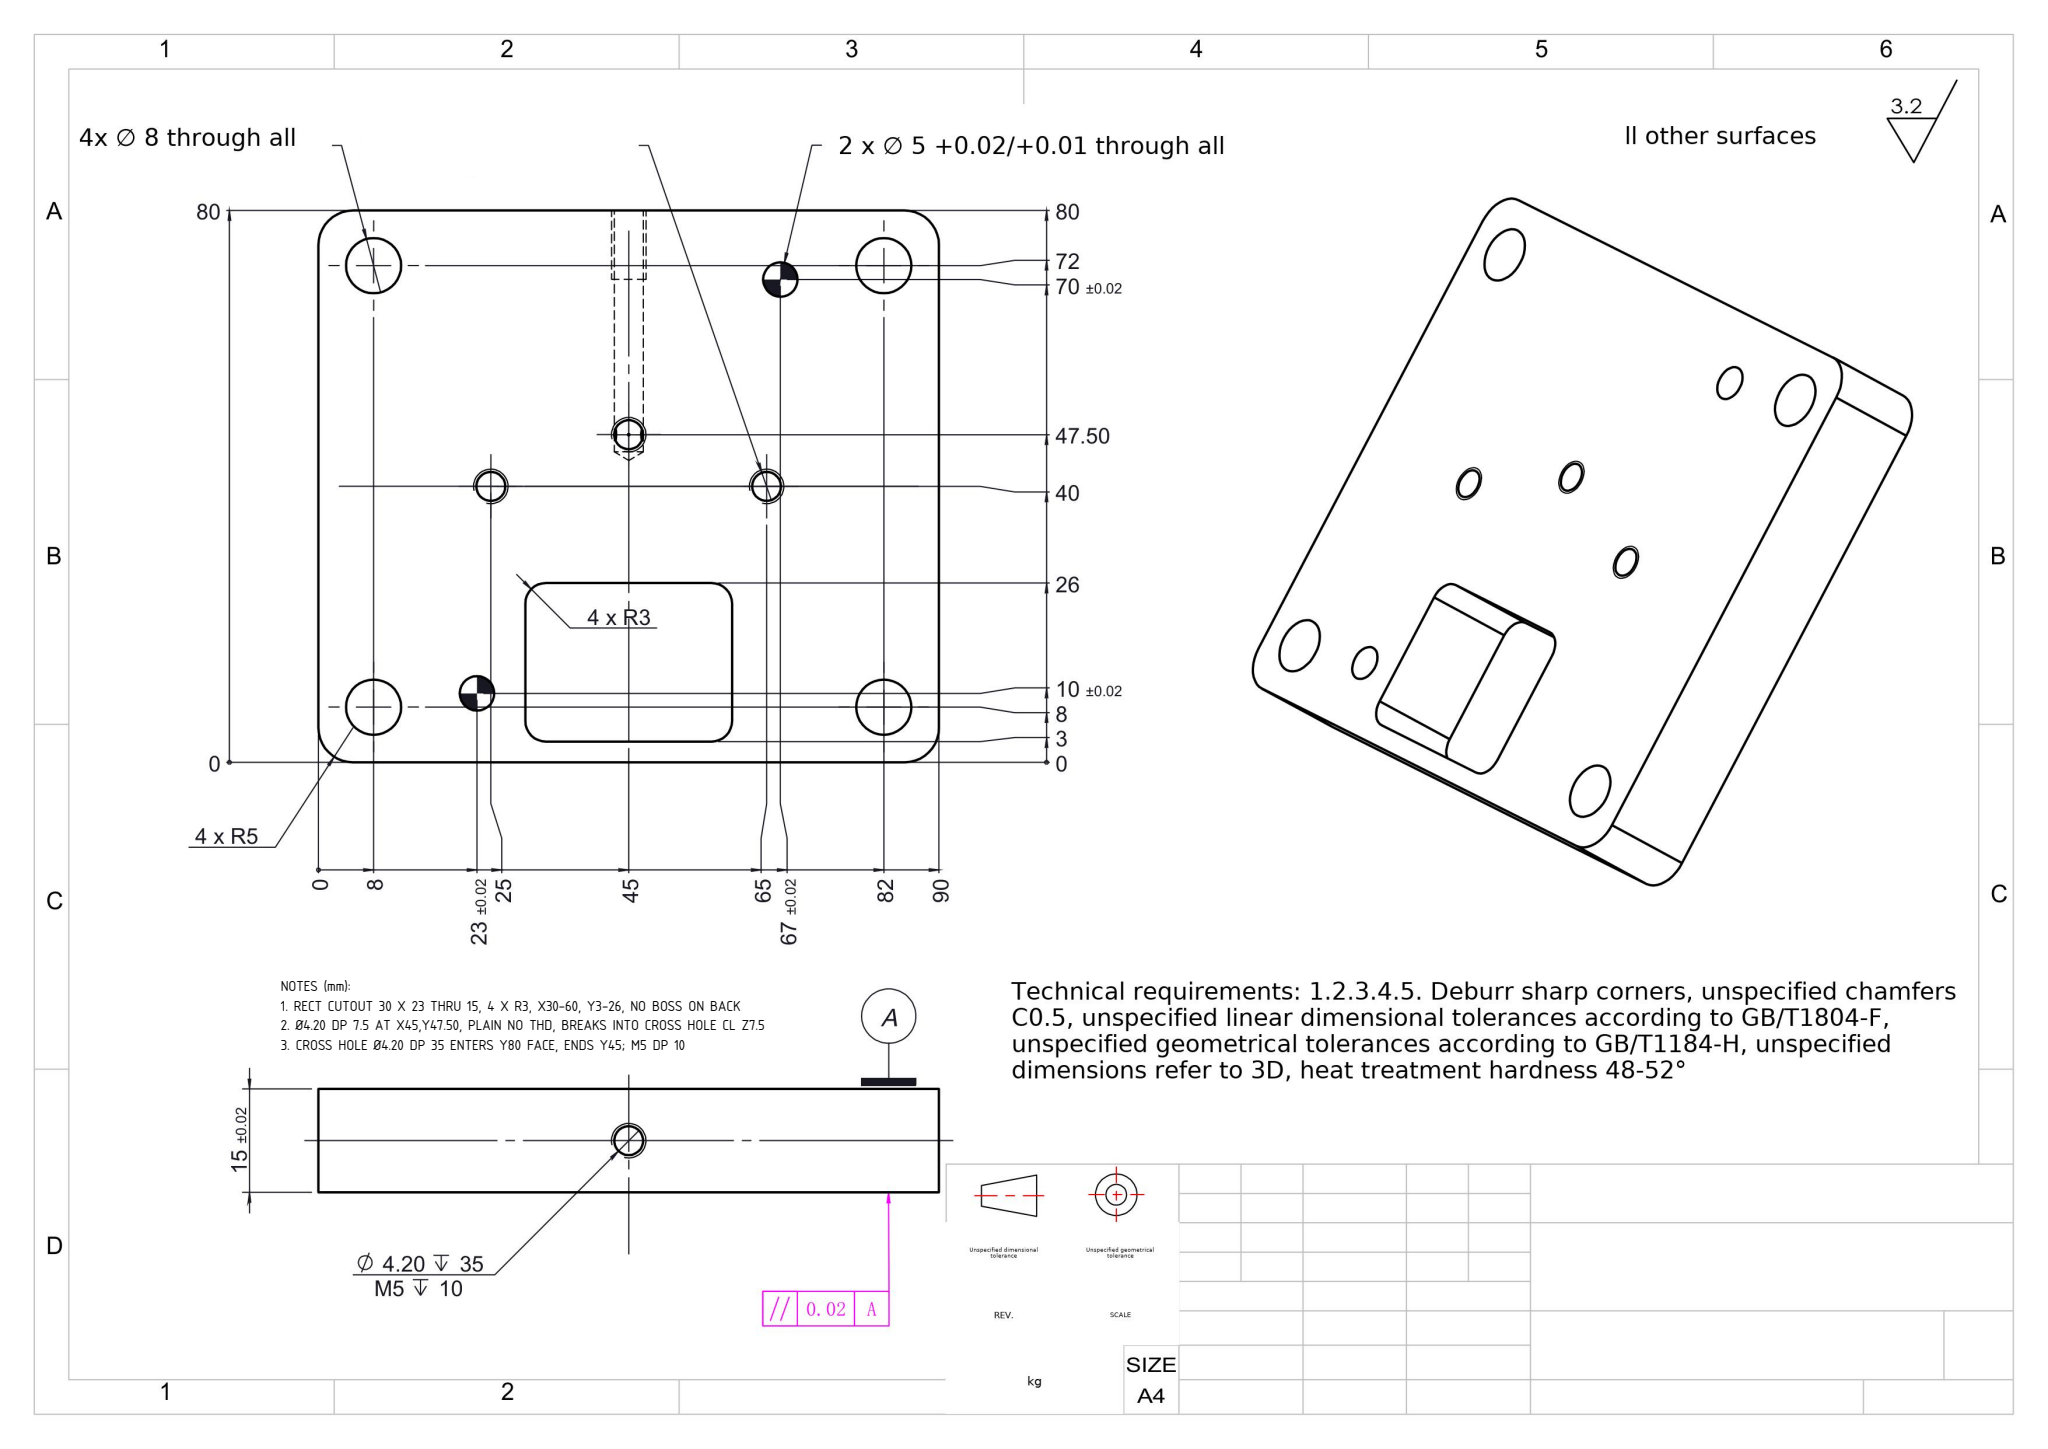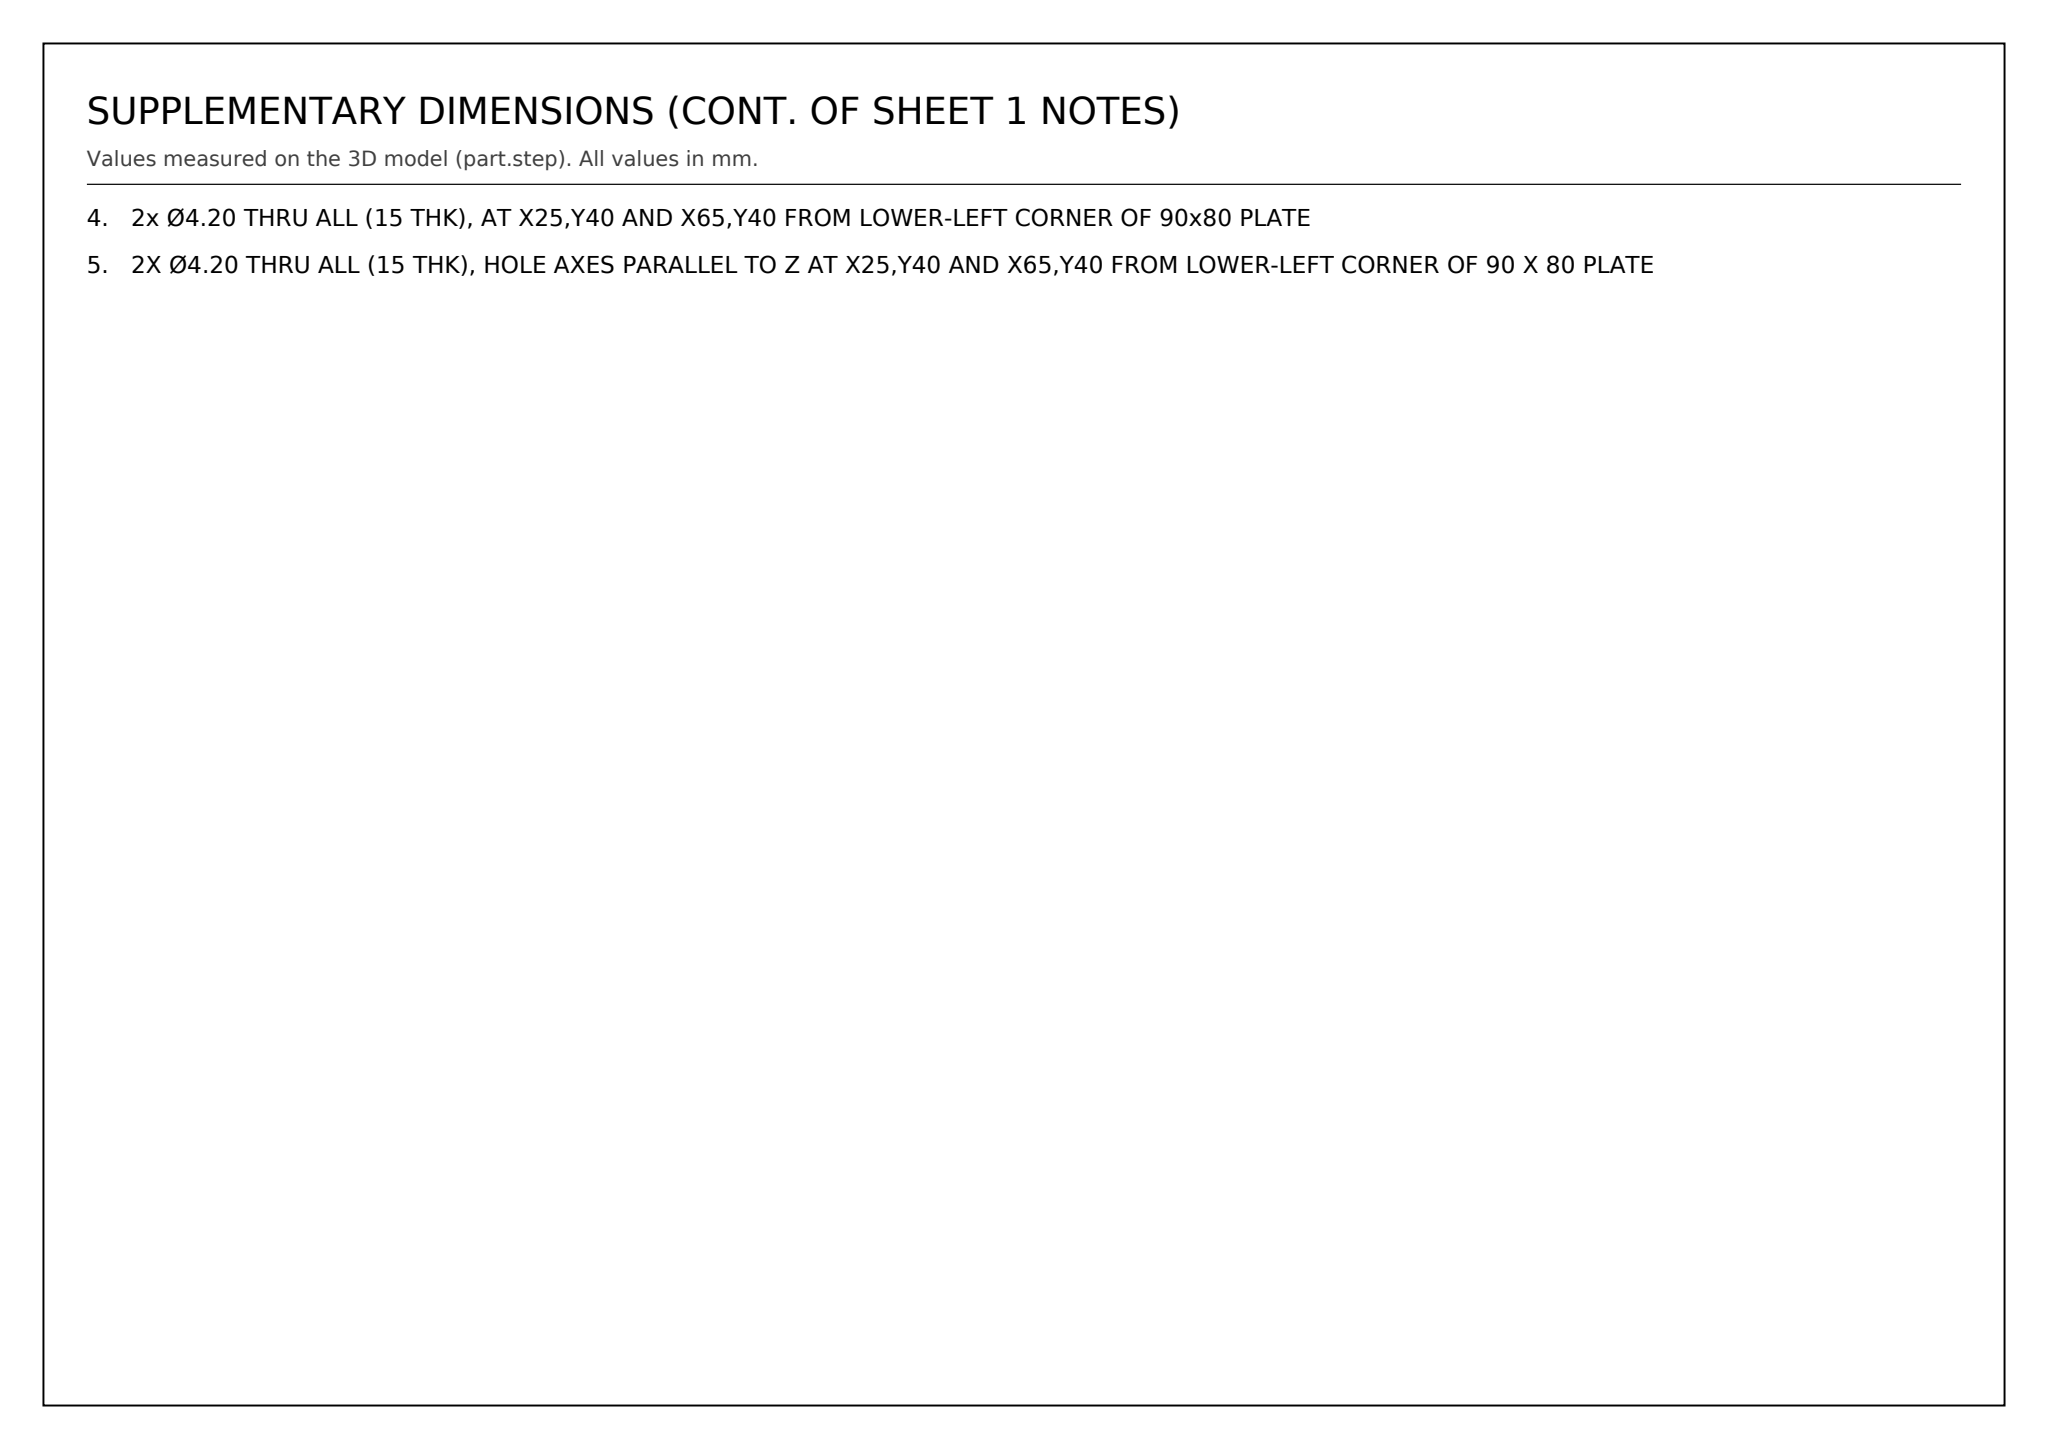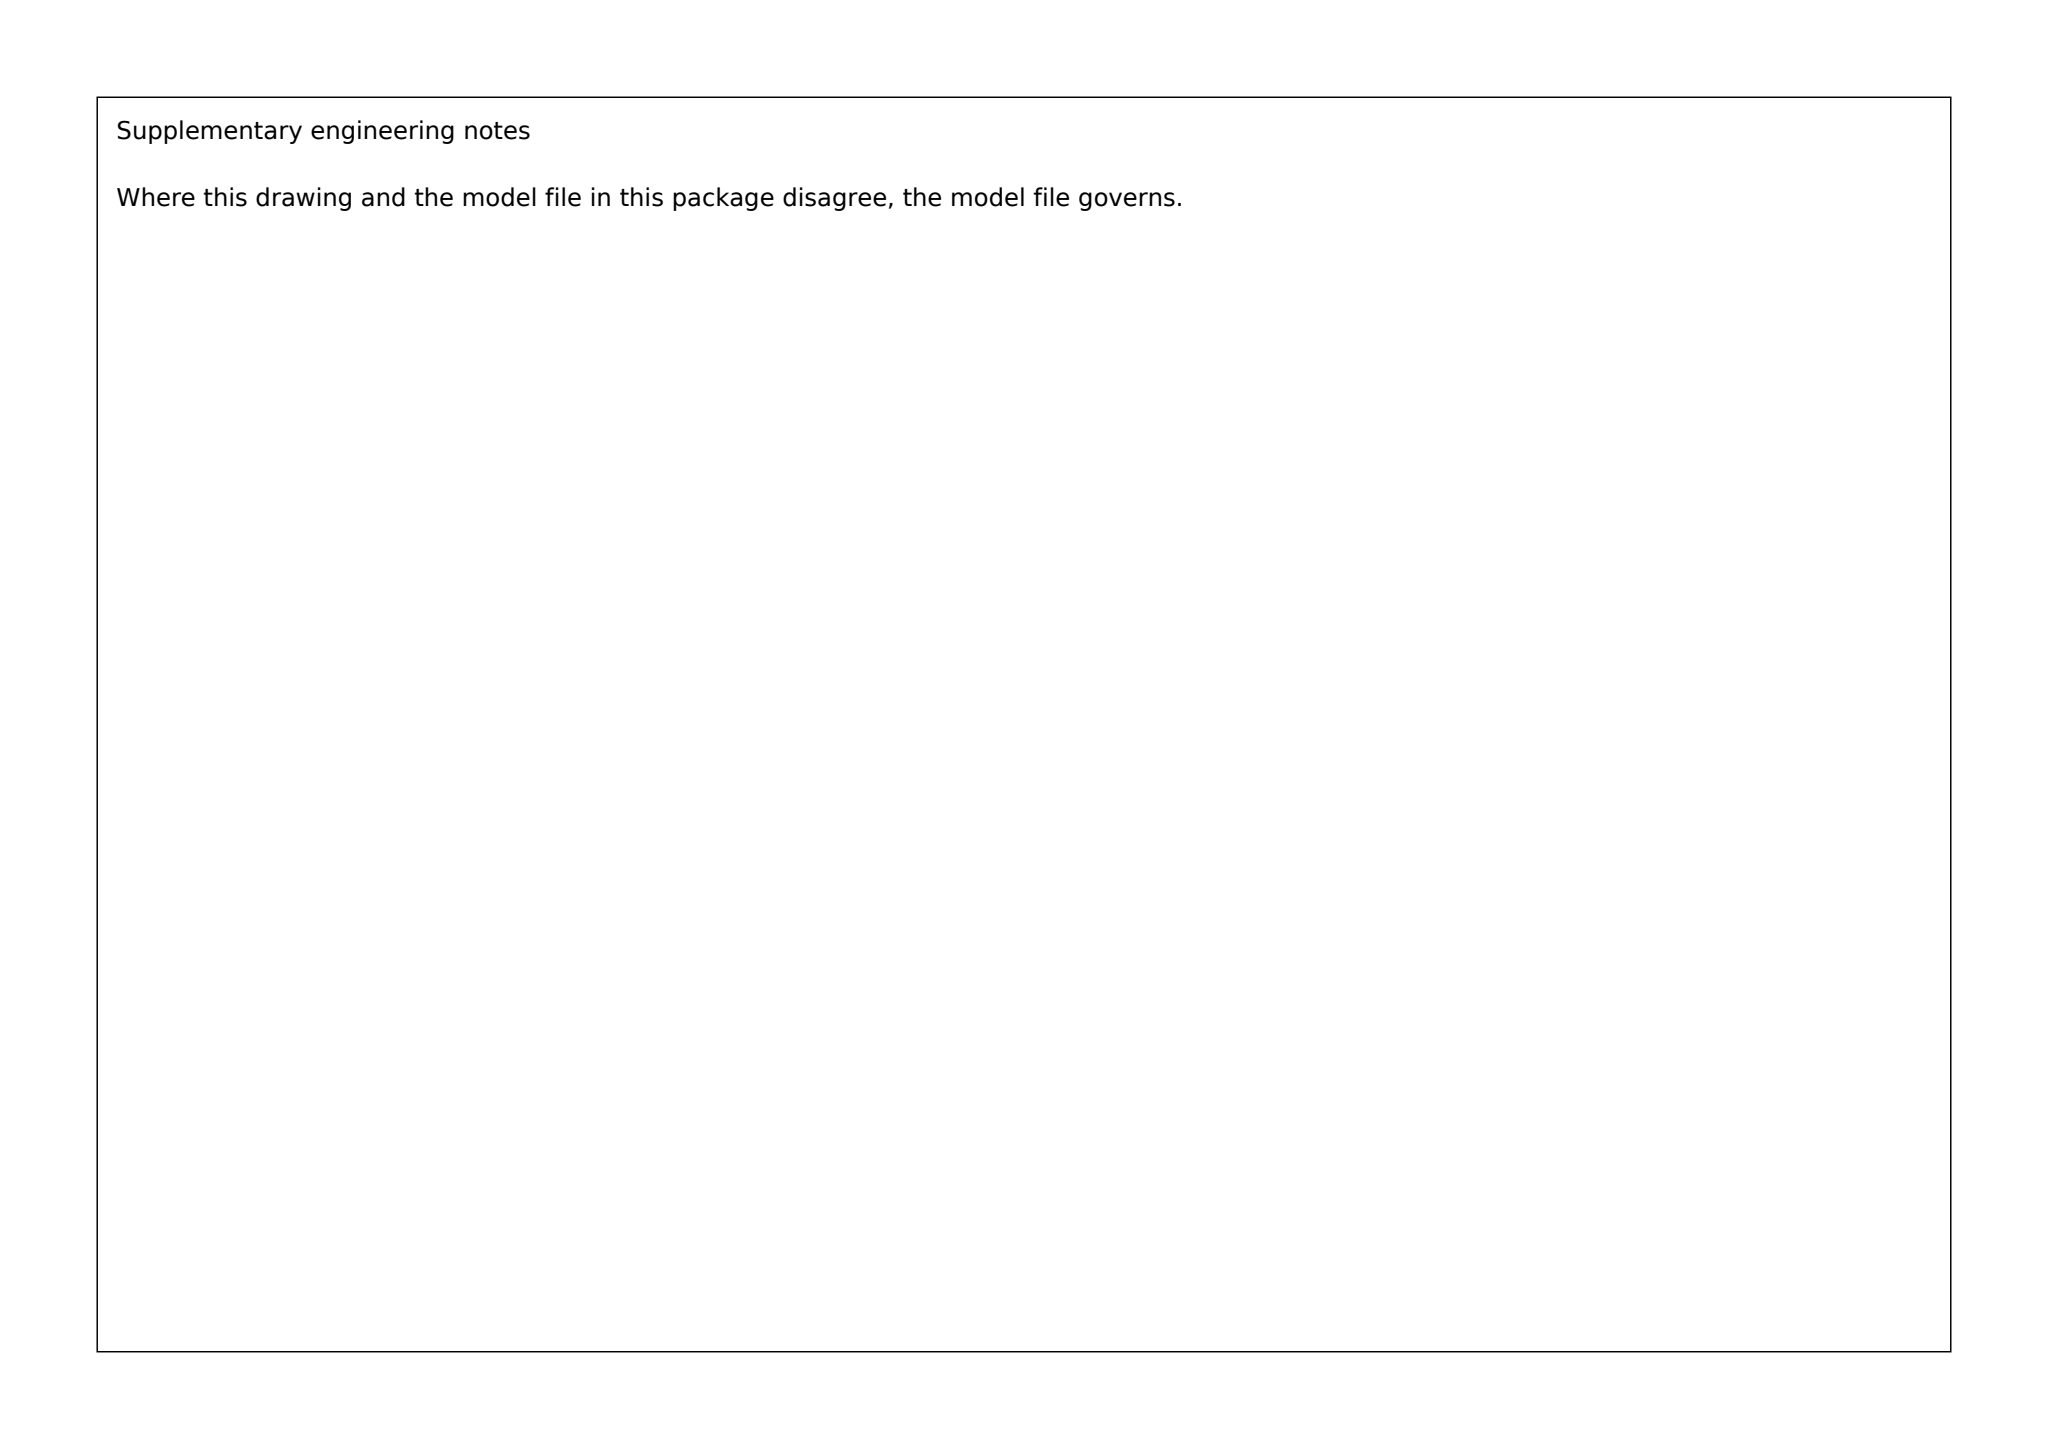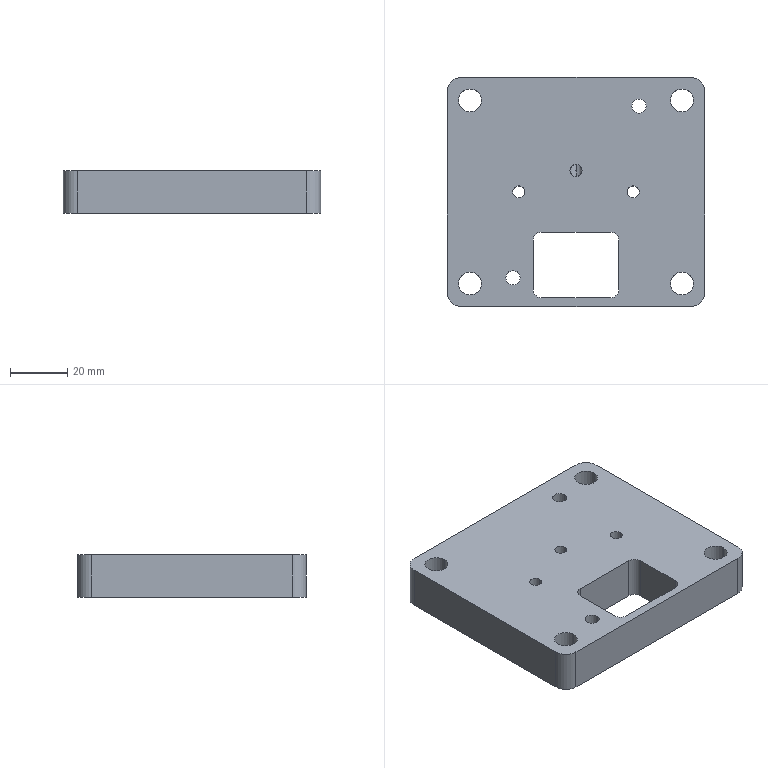Part | SolidWorks | mm | 1 solid | 48 faces | box 90 x 80 x 15 mm | volume 92853 mm3 | cylinder 31 | plane 10 | cone 7 | commonest cylinder face diameters 4.2 x11 8 x8 5 x4 10 x4 6 x4
Drawing notes:
RECT CUTOUT 30 X 23 THRU 15, 4 X R3, X30-60, Y3-26, NO BOSS ON BACK | from the solid: Planes x=30,60 & y=3,26; R3 (Ø6) corner cyls at (33,6),(33,23),(57,6),(57,23) len 15 = full thk; only z planes 0 and 15
Ø4.20 DP 7.5 AT X45,Y47.50, PLAIN NO THD, BREAKS INTO CROSS HOLE CL Z7.5 | from the solid: z-cyl Ø4.2 at [45,47.5] len 7.5 from top face z=15; y-axis Ø4.2 cross hole CL at z=7.5; 118° drill point ref dia 4.2; no thread geometry
CROSS HOLE Ø4.20 DP 35 ENTERS Y80 FACE, ENDS Y45; M5 DP 10 | from the solid: cyl dia4.2 axis y at (x=45, z=7.5), length 35; spans Y45-Y80 so Y47.50 Ø4.20 ↧7.5 Z-hole breaks into it (bbox Y=80)
2x Ø4.20 THRU ALL (15 THK), AT X25,Y40 AND X65,Y40 FROM LOWER-LEFT CORNER OF 90x80 PLATE | from the solid: cylinders[4.2,"z",[25.0,40.0,null],15.0] and [4.2,"z",[65.0,40.0,null],15.0]; bbox_xyz 90x80x15
2X Ø4.20 THRU ALL (15 THK), HOLE AXES PARALLEL TO Z AT X25,Y40 AND X65,Y40 FROM LOWER-LEFT CORNER OF 90 X 80 PLATE | from the solid: cylinders [4.2,"z",[25.0,40.0,null],15.0] and [4.2,"z",[65.0,40.0,null],15.0]; bbox_xyz 90x80x15
build123d program:
from build123d import *

# Parameters (mm, degrees)
SKETCH1_W                  = 90
SKETCH1_H                  = 80
BOSS_EXTRUDE1_DEPTH        = 15
SIZE_MM_DOWEL_PIN_HOLE_0_D = 5
F_8_0_8_DIAMETER_HOLE1_D   = 8
M5_TAPPED_HOLE1_D          = 4.2
M5_TAPPED_HOLE1_DEPTH      = 8.4
M5_TAPPED_HOLE1_TIP        = 1.262
M5_TAPPED_HOLE2_D          = 4.2
M5_TAPPED_HOLE2_DEPTH      = 35
M5_TAPPED_HOLE2_TIP        = 1.262
FILLET1_R                  = 5
M5_CLEARANCE_HOLE_1_D      = 5.5
SKETCH12_W                 = 30
SKETCH12_H                 = 23
CUT_EXTRUDE1_DEPTH         = 63.048
FILLET2_R                  = 3
M5_TAPPED_HOLE3_D          = 4.2


with BuildPart() as part:
    # Sketch1 → Boss-Extrude1 (new body)
    with BuildSketch(Plane.XY):
        Rectangle(SKETCH1_W, SKETCH1_H)
    extrude(amount=BOSS_EXTRUDE1_DEPTH)

    # Size mm Dowel Pin Hole 0 (through all)
    with Locations(Plane.XY.offset(15)):
        with Locations((-22, -30), (22, 30)):
            Hole(SIZE_MM_DOWEL_PIN_HOLE_0_D / 2)

    # 8.0 _8_ Diameter Hole1 (through all)
    with Locations(Plane.XY.offset(15)):
        with Locations((-37, 32), (37, 32), (37, -32), (-37, -32)):
            Hole(F_8_0_8_DIAMETER_HOLE1_D / 2)

    # M5 Tapped Hole1
    with Locations(Plane.XY.offset(15)):
        with Locations((0, 7.5)):
            Hole(M5_TAPPED_HOLE1_D / 2, depth=M5_TAPPED_HOLE1_DEPTH)
            with Locations((0, 0, -(M5_TAPPED_HOLE1_DEPTH + M5_TAPPED_HOLE1_TIP / 2))):  # 118° drill point
                Cone(0, M5_TAPPED_HOLE1_D / 2, M5_TAPPED_HOLE1_TIP, mode=Mode.SUBTRACT)

    # M5 Tapped Hole2
    with Locations(Plane(origin=(0, 40, 0), x_dir=(1, 0, 0), z_dir=(0, 1, 0))):
        with Locations((0, -7.5)):
            Hole(M5_TAPPED_HOLE2_D / 2, depth=M5_TAPPED_HOLE2_DEPTH)
            with Locations((0, 0, -(M5_TAPPED_HOLE2_DEPTH + M5_TAPPED_HOLE2_TIP / 2))):  # 118° drill point
                Cone(0, M5_TAPPED_HOLE2_D / 2, M5_TAPPED_HOLE2_TIP, mode=Mode.SUBTRACT)

    # Fillet1
    fillet1_edges = [part.edges().sort_by_distance(p)[0] for p in [
        (45, -40, 7.5),
        (-45, -40, 7.5),
        (-45, 40, 7.5),
        (45, 40, 7.5),
    ]]
    fillet(fillet1_edges, radius=FILLET1_R)

    # M5 Clearance Hole 1 (through all)
    with Locations(Plane.XY.offset(15)):
        with Locations((-10.094, -28), (9.906, -28)):
            Hole(M5_CLEARANCE_HOLE_1_D / 2)

    # Sketch12 → Cut-Extrude1 (cut, through all)
    with BuildSketch(Plane.XY.offset(15)):
        with Locations((0, -25.5)):
            Rectangle(SKETCH12_W, SKETCH12_H)
    extrude(amount=-CUT_EXTRUDE1_DEPTH, mode=Mode.SUBTRACT)

    # Fillet2
    fillet2_edges = [part.edges().sort_by_distance(p)[0] for p in [
        (-15, -37, 7.5),
        (-15, -14, 7.5),
        (15, -14, 7.5),
        (15, -37, 7.5),
    ]]
    fillet(fillet2_edges, radius=FILLET2_R)

    # M5 Tapped Hole3 (through all)
    with Locations(Plane.XY.offset(15)):
        with Locations((-20, 0), (20, 0)):
            Hole(M5_TAPPED_HOLE3_D / 2)


solid = part.part